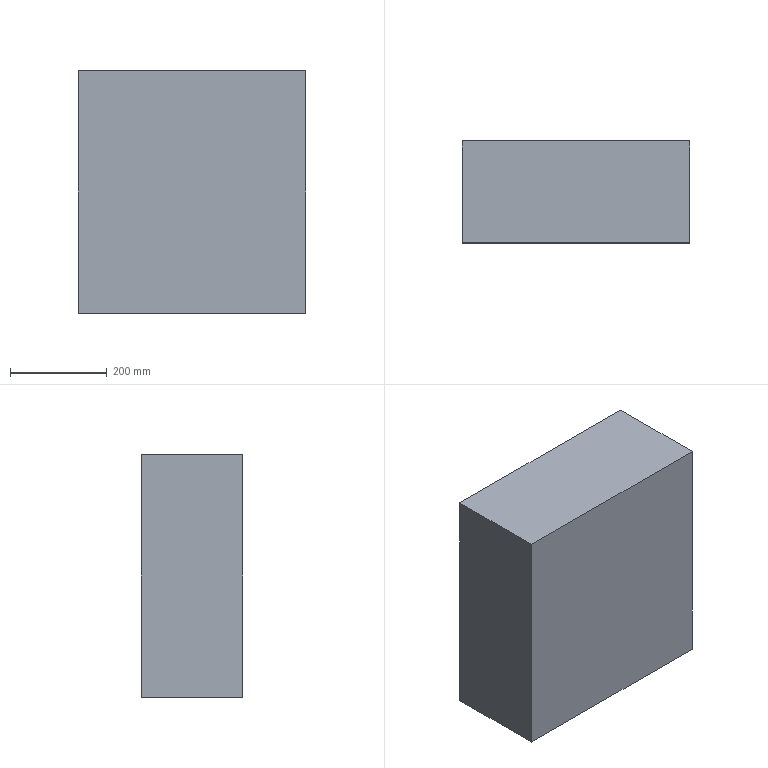Component | SolidWorks | CoolantTank-1 | 1 solid | 12 faces | box 470 x 210 x 500 mm | volume 5190000 mm3 | plane 12 | material 45
STEP:
#1=COLOUR_RGB('',0.7922,0.8196,0.9333);
#2=FILL_AREA_STYLE_COLOUR('',#1);
#3=FILL_AREA_STYLE('',(#2));
#4=SURFACE_STYLE_FILL_AREA(#3);
#5=SURFACE_SIDE_STYLE('',(#4));
#6=SURFACE_STYLE_USAGE(.BOTH.,#5);
#7=PRESENTATION_STYLE_ASSIGNMENT((#6));
#8=CARTESIAN_POINT('',(-12.591,-6.676,29.617));
#9=VERTEX_POINT('',#8);
#10=CARTESIAN_POINT('',(-12.591,-14.944,29.617));
#11=VERTEX_POINT('',#10);
#12=CARTESIAN_POINT('',(-12.591,-14.747,29.617));
#13=DIRECTION('',(-0.,-1.,0.));
#14=VECTOR('',#13,39.37);
#15=LINE('',#12,#14);
#16=EDGE_CURVE('',#9,#11,#15,.T.);
#17=ORIENTED_EDGE('',*,*,#16,.T.);
#18=CARTESIAN_POINT('',(-12.591,-14.944,49.302));
#19=VERTEX_POINT('',#18);
#20=CARTESIAN_POINT('',(-12.591,-14.944,49.302));
#21=DIRECTION('',(0.,0.,-1.));
#22=VECTOR('',#21,39.37);
#23=LINE('',#20,#22);
#24=EDGE_CURVE('',#19,#11,#23,.T.);
#25=ORIENTED_EDGE('',*,*,#24,.F.);
#26=CARTESIAN_POINT('',(-12.591,-6.676,49.302));
#27=VERTEX_POINT('',#26);
#28=CARTESIAN_POINT('',(-12.591,-14.747,49.302));
#29=DIRECTION('',(-0.,-1.,0.));
#30=VECTOR('',#29,39.37);
#31=LINE('',#28,#30);
#32=EDGE_CURVE('',#27,#19,#31,.T.);
#33=ORIENTED_EDGE('',*,*,#32,.F.);
#34=CARTESIAN_POINT('',(-12.591,-6.676,49.302));
#35=DIRECTION('',(0.,0.,-1.));
#36=VECTOR('',#35,39.37);
#37=LINE('',#34,#36);
#38=EDGE_CURVE('',#27,#9,#37,.T.);
#39=ORIENTED_EDGE('',*,*,#38,.T.);
#40=EDGE_LOOP('',(#17,#25,#33,#39));
#41=FACE_OUTER_BOUND('',#40,.T.);
#42=CARTESIAN_POINT('',(-12.591,-14.747,49.302));
#43=DIRECTION('',(1.,-0.,0.));
#44=DIRECTION('',(0.,1.,0.));
#45=AXIS2_PLACEMENT_3D('',#42,#43,#44);
#46=PLANE('',#45);
#47=ADVANCED_FACE('',(#41),#46,.F.);
#48=CARTESIAN_POINT('',(5.913,-14.944,29.617));
#49=VERTEX_POINT('',#48);
#50=CARTESIAN_POINT('',(5.716,-14.944,29.617));
#51=DIRECTION('',(1.,0.,0.));
#52=VECTOR('',#51,39.37);
#53=LINE('',#50,#52);
#54=EDGE_CURVE('',#11,#49,#53,.T.);
#55=ORIENTED_EDGE('',*,*,#54,.T.);
#56=CARTESIAN_POINT('',(5.913,-14.944,49.302));
#57=VERTEX_POINT('',#56);
#58=CARTESIAN_POINT('',(5.913,-14.944,49.302));
#59=DIRECTION('',(0.,0.,-1.));
#60=VECTOR('',#59,39.37);
#61=LINE('',#58,#60);
#62=EDGE_CURVE('',#57,#49,#61,.T.);
#63=ORIENTED_EDGE('',*,*,#62,.F.);
#64=CARTESIAN_POINT('',(5.716,-14.944,49.302));
#65=DIRECTION('',(1.,0.,0.));
#66=VECTOR('',#65,39.37);
#67=LINE('',#64,#66);
#68=EDGE_CURVE('',#19,#57,#67,.T.);
#69=ORIENTED_EDGE('',*,*,#68,.F.);
#70=ORIENTED_EDGE('',*,*,#24,.T.);
#71=EDGE_LOOP('',(#55,#63,#69,#70));
#72=FACE_OUTER_BOUND('',#71,.T.);
#73=CARTESIAN_POINT('',(5.716,-14.944,49.302));
#74=DIRECTION('',(-0.,1.,0.));
#75=DIRECTION('',(-1.,-0.,0.));
#76=AXIS2_PLACEMENT_3D('',#73,#74,#75);
#77=PLANE('',#76);
#78=ADVANCED_FACE('',(#72),#77,.F.);
#79=CARTESIAN_POINT('',(5.913,-6.676,29.617));
#80=VERTEX_POINT('',#79);
#81=CARTESIAN_POINT('',(5.913,-14.747,29.617));
#82=DIRECTION('',(0.,1.,0.));
#83=VECTOR('',#82,39.37);
#84=LINE('',#81,#83);
#85=EDGE_CURVE('',#49,#80,#84,.T.);
#86=ORIENTED_EDGE('',*,*,#85,.T.);
#87=CARTESIAN_POINT('',(5.913,-6.676,49.302));
#88=VERTEX_POINT('',#87);
#89=CARTESIAN_POINT('',(5.913,-6.676,49.302));
#90=DIRECTION('',(0.,0.,-1.));
#91=VECTOR('',#90,39.37);
#92=LINE('',#89,#91);
#93=EDGE_CURVE('',#88,#80,#92,.T.);
#94=ORIENTED_EDGE('',*,*,#93,.F.);
#95=CARTESIAN_POINT('',(5.913,-14.747,49.302));
#96=DIRECTION('',(0.,1.,0.));
#97=VECTOR('',#96,39.37);
#98=LINE('',#95,#97);
#99=EDGE_CURVE('',#57,#88,#98,.T.);
#100=ORIENTED_EDGE('',*,*,#99,.F.);
#101=ORIENTED_EDGE('',*,*,#62,.T.);
#102=EDGE_LOOP('',(#86,#94,#100,#101));
#103=FACE_OUTER_BOUND('',#102,.T.);
#104=CARTESIAN_POINT('',(5.913,-14.747,49.302));
#105=DIRECTION('',(-1.,0.,0.));
#106=DIRECTION('',(0.,0.,1.));
#107=AXIS2_PLACEMENT_3D('',#104,#105,#106);
#108=PLANE('',#107);
#109=ADVANCED_FACE('',(#103),#108,.F.);
#110=CARTESIAN_POINT('',(5.716,-6.676,29.617));
#111=DIRECTION('',(-1.,-0.,0.));
#112=VECTOR('',#111,39.37);
#113=LINE('',#110,#112);
#114=EDGE_CURVE('',#80,#9,#113,.T.);
#115=ORIENTED_EDGE('',*,*,#114,.T.);
#116=ORIENTED_EDGE('',*,*,#38,.F.);
#117=CARTESIAN_POINT('',(5.716,-6.676,49.302));
#118=DIRECTION('',(-1.,-0.,0.));
#119=VECTOR('',#118,39.37);
#120=LINE('',#117,#119);
#121=EDGE_CURVE('',#88,#27,#120,.T.);
#122=ORIENTED_EDGE('',*,*,#121,.F.);
#123=ORIENTED_EDGE('',*,*,#93,.T.);
#124=EDGE_LOOP('',(#115,#116,#122,#123));
#125=FACE_OUTER_BOUND('',#124,.T.);
#126=CARTESIAN_POINT('',(5.716,-6.676,49.302));
#127=DIRECTION('',(0.,-1.,0.));
#128=DIRECTION('',(1.,0.,0.));
#129=AXIS2_PLACEMENT_3D('',#126,#127,#128);
#130=PLANE('',#129);
#131=ADVANCED_FACE('',(#125),#130,.F.);
#132=ORIENTED_EDGE('',*,*,#32,.T.);
#133=ORIENTED_EDGE('',*,*,#68,.T.);
#134=ORIENTED_EDGE('',*,*,#99,.T.);
#135=ORIENTED_EDGE('',*,*,#121,.T.);
#136=EDGE_LOOP('',(#132,#133,#134,#135));
#137=FACE_OUTER_BOUND('',#136,.T.);
#138=CARTESIAN_POINT('',(-3.339,-10.81,49.302));
#139=DIRECTION('',(0.,0.,1.));
#140=DIRECTION('',(1.,0.,0.));
#141=AXIS2_PLACEMENT_3D('',#138,#139,#140);
#142=PLANE('',#141);
#143=ADVANCED_FACE('',(#137),#142,.T.);
#144=ORIENTED_EDGE('',*,*,#16,.F.);
#145=ORIENTED_EDGE('',*,*,#114,.F.);
#146=ORIENTED_EDGE('',*,*,#85,.F.);
#147=ORIENTED_EDGE('',*,*,#54,.F.);
#148=EDGE_LOOP('',(#144,#145,#146,#147));
#149=FACE_OUTER_BOUND('',#148,.T.);
#150=CARTESIAN_POINT('',(-3.339,-10.81,29.617));
#151=DIRECTION('',(0.,0.,1.));
#152=DIRECTION('',(1.,0.,0.));
#153=AXIS2_PLACEMENT_3D('',#150,#151,#152);
#154=PLANE('',#153);
#155=ADVANCED_FACE('',(#149),#154,.F.);
#156=CLOSED_SHELL('',(#47,#78,#109,#131,#143,#155));
#157=CARTESIAN_POINT('',(-12.394,-6.873,30.011));
#158=VERTEX_POINT('',#157);
#159=CARTESIAN_POINT('',(-12.394,-14.747,30.011));
#160=VERTEX_POINT('',#159);
#161=CARTESIAN_POINT('',(-12.394,-14.747,30.011));
#162=DIRECTION('',(-0.,-1.,0.));
#163=VECTOR('',#162,39.37);
#164=LINE('',#161,#163);
#165=EDGE_CURVE('',#158,#160,#164,.T.);
#166=ORIENTED_EDGE('',*,*,#165,.F.);
#167=CARTESIAN_POINT('',(-12.394,-6.873,48.908));
#168=VERTEX_POINT('',#167);
#169=CARTESIAN_POINT('',(-12.394,-6.873,48.908));
#170=DIRECTION('',(0.,0.,-1.));
#171=VECTOR('',#170,39.37);
#172=LINE('',#169,#171);
#173=EDGE_CURVE('',#168,#158,#172,.T.);
#174=ORIENTED_EDGE('',*,*,#173,.F.);
#175=CARTESIAN_POINT('',(-12.394,-14.747,48.908));
#176=VERTEX_POINT('',#175);
#177=CARTESIAN_POINT('',(-12.394,-14.747,48.908));
#178=DIRECTION('',(-0.,-1.,0.));
#179=VECTOR('',#178,39.37);
#180=LINE('',#177,#179);
#181=EDGE_CURVE('',#168,#176,#180,.T.);
#182=ORIENTED_EDGE('',*,*,#181,.T.);
#183=CARTESIAN_POINT('',(-12.394,-14.747,48.908));
#184=DIRECTION('',(0.,0.,-1.));
#185=VECTOR('',#184,39.37);
#186=LINE('',#183,#185);
#187=EDGE_CURVE('',#176,#160,#186,.T.);
#188=ORIENTED_EDGE('',*,*,#187,.T.);
#189=EDGE_LOOP('',(#166,#174,#182,#188));
#190=FACE_OUTER_BOUND('',#189,.T.);
#191=CARTESIAN_POINT('',(-12.394,-14.747,48.908));
#192=DIRECTION('',(1.,-0.,0.));
#193=DIRECTION('',(0.,1.,0.));
#194=AXIS2_PLACEMENT_3D('',#191,#192,#193);
#195=PLANE('',#194);
#196=ADVANCED_FACE('',(#190),#195,.T.);
#197=CARTESIAN_POINT('',(5.716,-14.747,30.011));
#198=VERTEX_POINT('',#197);
#199=CARTESIAN_POINT('',(5.716,-14.747,30.011));
#200=DIRECTION('',(1.,0.,0.));
#201=VECTOR('',#200,39.37);
#202=LINE('',#199,#201);
#203=EDGE_CURVE('',#160,#198,#202,.T.);
#204=ORIENTED_EDGE('',*,*,#203,.F.);
#205=ORIENTED_EDGE('',*,*,#187,.F.);
#206=CARTESIAN_POINT('',(5.716,-14.747,48.908));
#207=VERTEX_POINT('',#206);
#208=CARTESIAN_POINT('',(5.716,-14.747,48.908));
#209=DIRECTION('',(1.,0.,0.));
#210=VECTOR('',#209,39.37);
#211=LINE('',#208,#210);
#212=EDGE_CURVE('',#176,#207,#211,.T.);
#213=ORIENTED_EDGE('',*,*,#212,.T.);
#214=CARTESIAN_POINT('',(5.716,-14.747,48.908));
#215=DIRECTION('',(0.,0.,-1.));
#216=VECTOR('',#215,39.37);
#217=LINE('',#214,#216);
#218=EDGE_CURVE('',#207,#198,#217,.T.);
#219=ORIENTED_EDGE('',*,*,#218,.T.);
#220=EDGE_LOOP('',(#204,#205,#213,#219));
#221=FACE_OUTER_BOUND('',#220,.T.);
#222=CARTESIAN_POINT('',(5.716,-14.747,48.908));
#223=DIRECTION('',(-0.,1.,0.));
#224=DIRECTION('',(-1.,-0.,0.));
#225=AXIS2_PLACEMENT_3D('',#222,#223,#224);
#226=PLANE('',#225);
#227=ADVANCED_FACE('',(#221),#226,.T.);
#228=CARTESIAN_POINT('',(5.716,-6.873,30.011));
#229=VERTEX_POINT('',#228);
#230=CARTESIAN_POINT('',(5.716,-14.747,30.011));
#231=DIRECTION('',(0.,1.,0.));
#232=VECTOR('',#231,39.37);
#233=LINE('',#230,#232);
#234=EDGE_CURVE('',#198,#229,#233,.T.);
#235=ORIENTED_EDGE('',*,*,#234,.F.);
#236=ORIENTED_EDGE('',*,*,#218,.F.);
#237=CARTESIAN_POINT('',(5.716,-6.873,48.908));
#238=VERTEX_POINT('',#237);
#239=CARTESIAN_POINT('',(5.716,-14.747,48.908));
#240=DIRECTION('',(0.,1.,0.));
#241=VECTOR('',#240,39.37);
#242=LINE('',#239,#241);
#243=EDGE_CURVE('',#207,#238,#242,.T.);
#244=ORIENTED_EDGE('',*,*,#243,.T.);
#245=CARTESIAN_POINT('',(5.716,-6.873,48.908));
#246=DIRECTION('',(0.,0.,-1.));
#247=VECTOR('',#246,39.37);
#248=LINE('',#245,#247);
#249=EDGE_CURVE('',#238,#229,#248,.T.);
#250=ORIENTED_EDGE('',*,*,#249,.T.);
#251=EDGE_LOOP('',(#235,#236,#244,#250));
#252=FACE_OUTER_BOUND('',#251,.T.);
#253=CARTESIAN_POINT('',(5.716,-14.747,48.908));
#254=DIRECTION('',(-1.,0.,0.));
#255=DIRECTION('',(0.,0.,1.));
#256=AXIS2_PLACEMENT_3D('',#253,#254,#255);
#257=PLANE('',#256);
#258=ADVANCED_FACE('',(#252),#257,.T.);
#259=CARTESIAN_POINT('',(5.716,-6.873,30.011));
#260=DIRECTION('',(-1.,-0.,0.));
#261=VECTOR('',#260,39.37);
#262=LINE('',#259,#261);
#263=EDGE_CURVE('',#229,#158,#262,.T.);
#264=ORIENTED_EDGE('',*,*,#263,.F.);
#265=ORIENTED_EDGE('',*,*,#249,.F.);
#266=CARTESIAN_POINT('',(5.716,-6.873,48.908));
#267=DIRECTION('',(-1.,-0.,0.));
#268=VECTOR('',#267,39.37);
#269=LINE('',#266,#268);
#270=EDGE_CURVE('',#238,#168,#269,.T.);
#271=ORIENTED_EDGE('',*,*,#270,.T.);
#272=ORIENTED_EDGE('',*,*,#173,.T.);
#273=EDGE_LOOP('',(#264,#265,#271,#272));
#274=FACE_OUTER_BOUND('',#273,.T.);
#275=CARTESIAN_POINT('',(5.716,-6.873,48.908));
#276=DIRECTION('',(0.,-1.,0.));
#277=DIRECTION('',(1.,0.,0.));
#278=AXIS2_PLACEMENT_3D('',#275,#276,#277);
#279=PLANE('',#278);
#280=ADVANCED_FACE('',(#274),#279,.T.);
#281=ORIENTED_EDGE('',*,*,#181,.F.);
#282=ORIENTED_EDGE('',*,*,#270,.F.);
#283=ORIENTED_EDGE('',*,*,#243,.F.);
#284=ORIENTED_EDGE('',*,*,#212,.F.);
#285=EDGE_LOOP('',(#281,#282,#283,#284));
#286=FACE_OUTER_BOUND('',#285,.T.);
#287=CARTESIAN_POINT('',(-3.339,-10.81,48.908));
#288=DIRECTION('',(0.,0.,1.));
#289=DIRECTION('',(1.,0.,0.));
#290=AXIS2_PLACEMENT_3D('',#287,#288,#289);
#291=PLANE('',#290);
#292=ADVANCED_FACE('',(#286),#291,.F.);
#293=ORIENTED_EDGE('',*,*,#165,.T.);
#294=ORIENTED_EDGE('',*,*,#203,.T.);
#295=ORIENTED_EDGE('',*,*,#234,.T.);
#296=ORIENTED_EDGE('',*,*,#263,.T.);
#297=EDGE_LOOP('',(#293,#294,#295,#296));
#298=FACE_OUTER_BOUND('',#297,.T.);
#299=CARTESIAN_POINT('',(-3.339,-10.81,30.011));
#300=DIRECTION('',(0.,0.,1.));
#301=DIRECTION('',(1.,0.,0.));
#302=AXIS2_PLACEMENT_3D('',#299,#300,#301);
#303=PLANE('',#302);
#304=ADVANCED_FACE('',(#298),#303,.T.);
#305=CLOSED_SHELL('',(#196,#227,#258,#280,#292,#304));
#306=ORIENTED_CLOSED_SHELL('',*,#305,.F.);
#307=BREP_WITH_VOIDS('',#156,(#306));
#308=STYLED_ITEM('',(#7),#307);
#309=(LENGTH_UNIT()NAMED_UNIT(*)SI_UNIT($,.METRE.));
#310=LENGTH_MEASURE_WITH_UNIT(LENGTH_MEASURE(0.0254),#309);
#311=DIMENSIONAL_EXPONENTS(1.,0.,0.,0.,0.,0.,0.);
#312=(CONVERSION_BASED_UNIT('',#310)LENGTH_UNIT()NAMED_UNIT(#311));
#313=UNCERTAINTY_MEASURE_WITH_UNIT(LENGTH_MEASURE(0.00001),#312,'','');
#314=(NAMED_UNIT(*)PLANE_ANGLE_UNIT()SI_UNIT($,.RADIAN.));
#315=(NAMED_UNIT(*)SI_UNIT($,.STERADIAN.)SOLID_ANGLE_UNIT());
#316=(GEOMETRIC_REPRESENTATION_CONTEXT(3)GLOBAL_UNCERTAINTY_ASSIGNED_CONTEXT((#313))GLOBAL_UNIT_ASSIGNED_CONTEXT((#312,#314,#315))REPRESENTATION_CONTEXT('',''));
#317=MECHANICAL_DESIGN_GEOMETRIC_PRESENTATION_REPRESENTATION('',(#308),#316);
#318=PRESENTATION_LAYER_ASSIGNMENT('','',(#308));
#319=CARTESIAN_POINT('',(0.,0.,0.));
#320=DIRECTION('',(0.,0.,1.));
#321=DIRECTION('',(1.,0.,0.));
#322=AXIS2_PLACEMENT_3D('',#319,#320,#321);
#323=(LENGTH_UNIT()NAMED_UNIT(*)SI_UNIT($,.METRE.));
#324=LENGTH_MEASURE_WITH_UNIT(LENGTH_MEASURE(0.0254),#323);
#325=DIMENSIONAL_EXPONENTS(1.,0.,0.,0.,0.,0.,0.);
#326=(CONVERSION_BASED_UNIT('',#324)LENGTH_UNIT()NAMED_UNIT(#325));
#327=UNCERTAINTY_MEASURE_WITH_UNIT(LENGTH_MEASURE(0.00001),#326,'','');
#328=(NAMED_UNIT(*)PLANE_ANGLE_UNIT()SI_UNIT($,.RADIAN.));
#329=(NAMED_UNIT(*)SI_UNIT($,.STERADIAN.)SOLID_ANGLE_UNIT());
#330=(GEOMETRIC_REPRESENTATION_CONTEXT(3)GLOBAL_UNCERTAINTY_ASSIGNED_CONTEXT((#327))GLOBAL_UNIT_ASSIGNED_CONTEXT((#326,#328,#329))REPRESENTATION_CONTEXT('',''));
#331=ADVANCED_BREP_SHAPE_REPRESENTATION('',(#307,#322),#330);